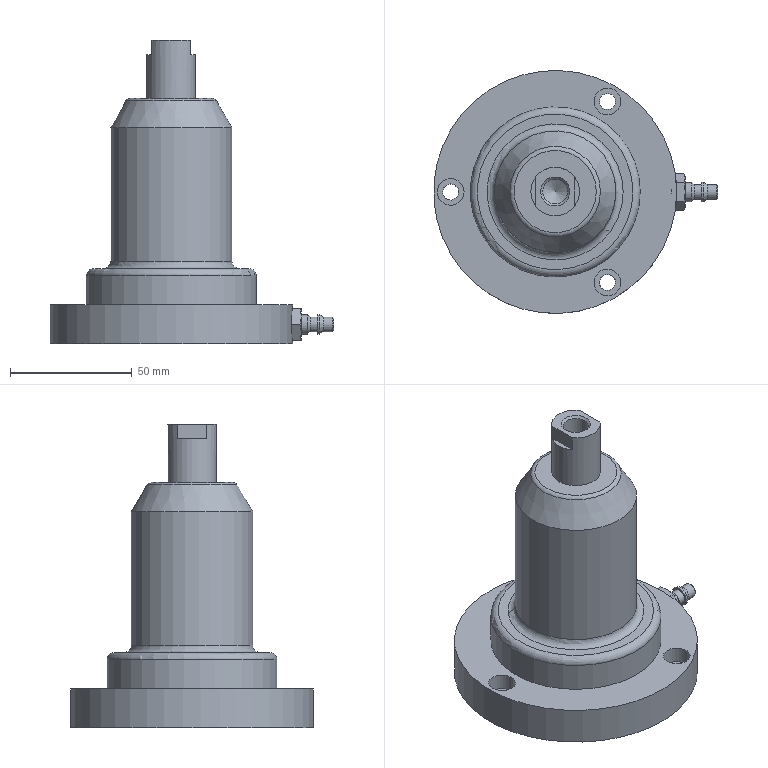Assembly | NX | mm | 14 component files | 14 solids | 268 faces | box 117 x 100 x 125 mm | volume 262783 mm3 | plane 112 | cylinder 78 | cone 41 | torus 32 | spline 5 | commonest cylinder face diameters 6 x20 10 x13 11 x9 40 x6 7 x6 8 x3 6.6 x3 34 x2
Bill of materials:
unnamed part 1 | 1 |  | Plain annular ring with a rectangular cross-section; its axial height is about the same as its radial wall width, so it is thicker than a typical flat washer.
unnamed part 2 | 1 |  | Flanged cylindrical bushing with a through bore. The main cylindrical body ends in a conical chamfered top, and a wider round-edged flange sits at the base, with a small fillet or step where the body meets the flange.
unnamed part 3 | 1 |  | Long slender tubular shaft standing on a flanged base. The base has a circumferential groove between two flange lips, and the top end has a stepped section with at least one flat. A bore opens at the top end.
unnamed part 4 | 1 |  | Thin flat ring with a narrow radial width and small axial thickness, like a washer or shim.
unnamed part 5 | 1 |  | Cylindrical helical coil spring of round wire with constant coil diameter, about 8 active coils with open pitch, and closed end coils.
unnamed part 6 | 6 |  | Solid stepped cylindrical pin: a short larger-diameter base cylinder topped by a smaller-diameter, longer shank with a chamfered free end.
unnamed part 7 | 1 |  | Axisymmetric tubular fitting-like body with a hexagonal collar. A long plain cylinder with a chamfered end extends on one side. On the other side is a stepped spigot: a cylinder, a taper down to a neck, a conical barb-like ridge, and a chamfered nose. A through bore runs along the axis.
unnamed part 8 | 1 |  | Thick circular disk or flange with a short raised central boss. The boss face has a shallow circular recess with a small central conical or countersunk hole. Nine axial through holes run through the disk: six on an inner bolt circle and three on an outer radius. One radial side hole with a spotface or counterbore enters the cylindrical edge.
unnamed part 9 | 1 |  | Flat annular ring or washer with a moderately wide radial width and a uniform rectangular cross-section.
Mates:
1. fix | End_Cap 1 component
2. concentric | End_Cap_Seal 1 arc | End_Cap 1 edge
3. concentric | Air_Cylinder 1 edge | End_Cap 1 arc
4. touch align | Air_Cylinder 1 face | End_Cap 1 face
5. concentric | Piston_Seal 1 arc | Piston_Rod 1 edge
6. touch align | SPRING_CYLINDER_COMPRESSION_1 1 datumaxis | Air_Cylinder 1 face
7. touch align | SPRING_CYLINDER_COMPRESSION_1 1 face | Air_Cylinder 1 face
8. touch align | Piston_Rod 1 face | Air_Cylinder 1 face
9. concentric | Tube_Seal 1 arc | End_Cap 1 edge
10. concentric | Tube_Connector 1 arc | Tube_Seal 1 edge
11. concentric | Hex_Socket_Screw_M6x10 6 edge | End_Cap 1 edge
12. bond | End_Cap 1 component | assembly component
13. bond | Hex_Socket_Screw_M6x10 6 component | assembly component
14. bond | Hex_Socket_Screw_M6x10 5 component | assembly component
15. bond | Hex_Socket_Screw_M6x10 4 component | assembly component
16. bond | Hex_Socket_Screw_M6x10 3 component | assembly component
17. bond | Hex_Socket_Screw_M6x10 2 component | assembly component
18. bond | Hex_Socket_Screw_M6x10 1 component | assembly component
19. circular | assembly datumaxis | assembly cartesiancoordinatesystem | assembly cartesiancoordinatesystem | assembly cartesiancoordinatesystem | assembly cartesiancoordinatesystem | assembly cartesiancoordinatesystem | assembly cartesiancoordinatesystem